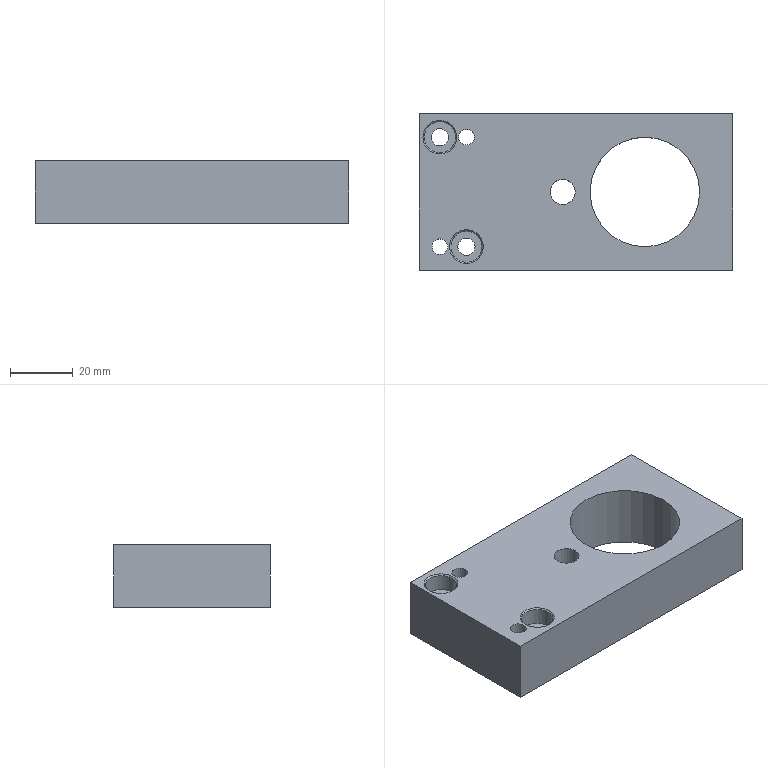Component | NX | DRILL_JIG_PLATE | 1 solid | 20 faces | volume 77373 mm3 | plane 8 | cylinder 8 | cone 4 | commonest cylinder face diameters 5.5 x2 10 x2 5 x2 35 x1 8 x1